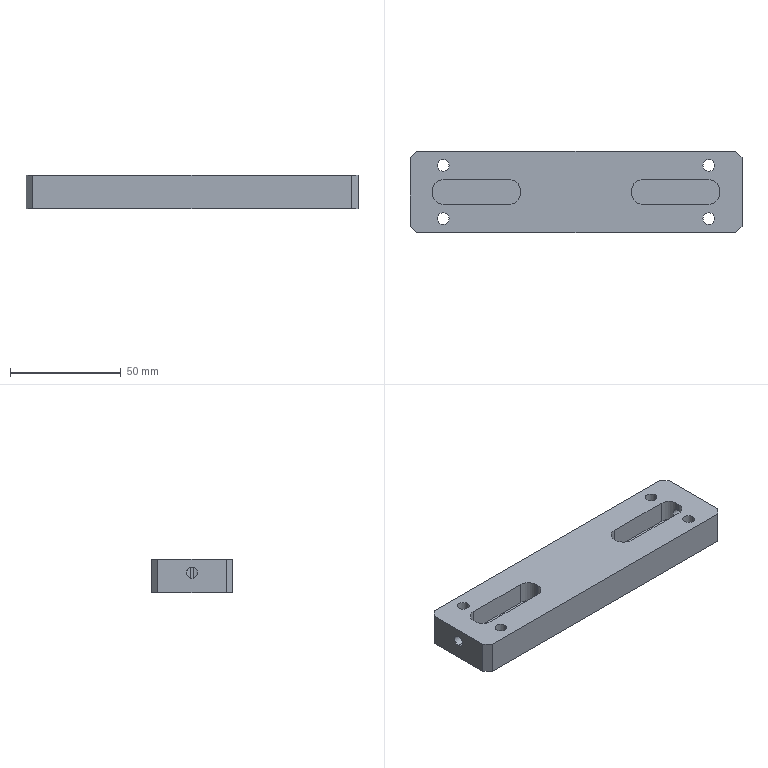Component | SolidWorks | --MA18S20041JR-SHuangGWAdjustingFixingBlock1-2 | 1 solid | 54 faces | box 150 x 37 x 15 mm | volume 71602 mm3 | cylinder 28 | plane 26 | commonest cylinder face diameters 10 x16 5.3 x8 5 x4
build123d program:
from build123d import *

# Parameters (mm, degrees)
SKETCH1_W                                            = 150
SKETCH1_H                                            = 37
BOSS_EXTRUDE1_DEPTH                                  = 15
SKETCH2_W                                            = 40
SKETCH2_H                                            = 11
CUT_EXTRUDE1_DEPTH                                   = 10
FILLET1_R                                            = 5
FILLET2_R                                            = 5
HOLE_SIZE_ACCORDING_TO_THE_TYPE_OF_HEXAG_D           = 5.3
HOLE_SIZE_ACCORDING_TO_THE_TYPE_OF_HEXAG_CBORE_D     = 10
HOLE_SIZE_ACCORDING_TO_THE_TYPE_OF_HEXAG_CBORE_DEPTH = 5.7
M6_TAPPED_HOLE1_D                                    = 5
M6_TAPPED_HOLE1_DEPTH                                = 15
M6_TAPPED_HOLE1_TIP                                  = 1.502
M6_TAPPED_HOLE2_D                                    = 5
M6_TAPPED_HOLE2_DEPTH                                = 15
M6_TAPPED_HOLE2_TIP                                  = 1.502
CHAMFER1_SIZE                                        = 3


with BuildPart() as part:
    # Sketch1 → Boss-Extrude1 (new body)
    with BuildSketch(Plane.XY):
        with Locations((75, 18.5)):
            Rectangle(SKETCH1_W, SKETCH1_H)
    extrude(amount=BOSS_EXTRUDE1_DEPTH)

    # Sketch2 → Cut-Extrude1 (cut)
    with BuildSketch(Plane(origin=(0, 0, 0), x_dir=(-1, 0, 0), z_dir=(0, 0, -1))):
        with Locations((-120, 18.5)):
            Rectangle(SKETCH2_W, SKETCH2_H)
        with Locations((-30, 18.5)):
            Rectangle(SKETCH2_W, SKETCH2_H)
    extrude(amount=-CUT_EXTRUDE1_DEPTH, mode=Mode.SUBTRACT)

    # Fillet1
    fillet1_edges = [part.edges().sort_by_distance(p)[0] for p in [
        (100, 24, 5),
        (100, 13, 5),
    ]]
    fillet(fillet1_edges, radius=FILLET1_R)

    # Fillet2
    fillet2_edges = [part.edges().sort_by_distance(p)[0] for p in [
        (140, 13, 5),
        (140, 24, 5),
        (50, 13, 5),
        (50, 24, 5),
        (10, 24, 5),
        (10, 13, 5),
    ]]
    fillet(fillet2_edges, radius=FILLET2_R)

    # Hole Size according to the type of Hexag (through all)
    with Locations(Plane.XY.offset(15)):
        with Locations((15, 30.5), (135, 30.5), (15, 6.5), (135, 6.5)):
            CounterBoreHole(HOLE_SIZE_ACCORDING_TO_THE_TYPE_OF_HEXAG_D / 2, HOLE_SIZE_ACCORDING_TO_THE_TYPE_OF_HEXAG_CBORE_D / 2, HOLE_SIZE_ACCORDING_TO_THE_TYPE_OF_HEXAG_CBORE_DEPTH)

    # M6 Tapped Hole1
    with Locations(Plane.ZY):
        with Locations((6, 18.5)):
            Hole(M6_TAPPED_HOLE1_D / 2, depth=M6_TAPPED_HOLE1_DEPTH)
            with Locations((0, 0, -(M6_TAPPED_HOLE1_DEPTH + M6_TAPPED_HOLE1_TIP / 2))):  # 118° drill point
                Cone(0, M6_TAPPED_HOLE1_D / 2, M6_TAPPED_HOLE1_TIP, mode=Mode.SUBTRACT)

    # M6 Tapped Hole2
    with Locations(Plane(origin=(150, 0, 0), x_dir=(0, 0, -1), z_dir=(1, 0, 0))):
        with Locations((-6, 18.5)):
            Hole(M6_TAPPED_HOLE2_D / 2, depth=M6_TAPPED_HOLE2_DEPTH)
            with Locations((0, 0, -(M6_TAPPED_HOLE2_DEPTH + M6_TAPPED_HOLE2_TIP / 2))):  # 118° drill point
                Cone(0, M6_TAPPED_HOLE2_D / 2, M6_TAPPED_HOLE2_TIP, mode=Mode.SUBTRACT)

    # Chamfer1
    chamfer1_edges = [part.edges().sort_by_distance(p)[0] for p in [
        (0, 37, 7.5),
        (150, 37, 7.5),
        (150, 0, 7.5),
        (0, 0, 7.5),
    ]]
    chamfer(chamfer1_edges, length=CHAMFER1_SIZE)


solid = part.part

# Placed as in the assembly
solid = solid.moved(Location((-2.956, 57.199, 0), (180, 0, 0)))